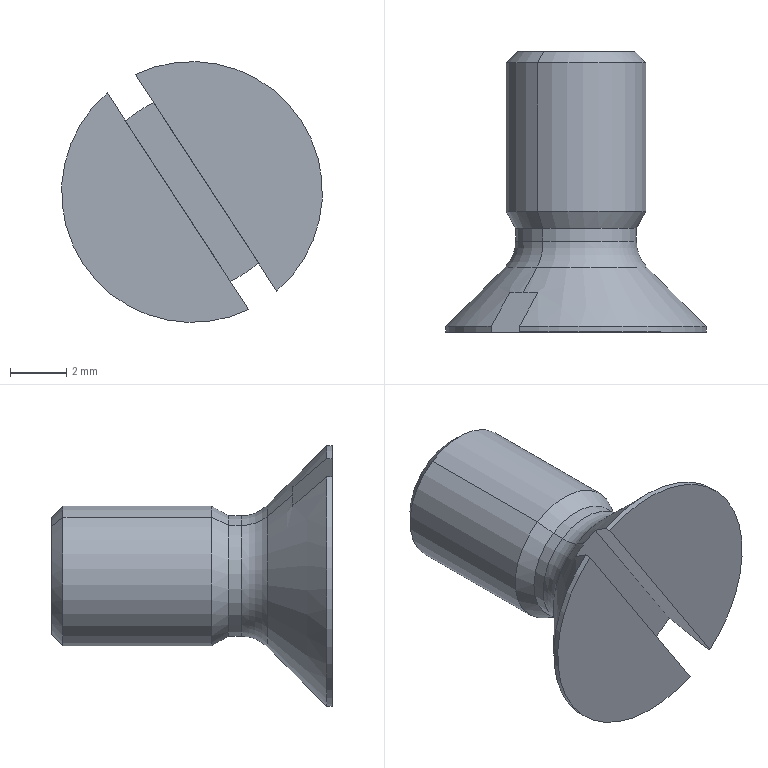Component | NX | SLOTTED_COUNTERSUNK_SCREW_M5X10_2 | 1 solid | 20 faces | volume 231 mm3 | cone 6 | cylinder 6 | plane 6 | torus 2 | commonest cylinder face diameters 5 x2 4.307 x2 9.3 x2